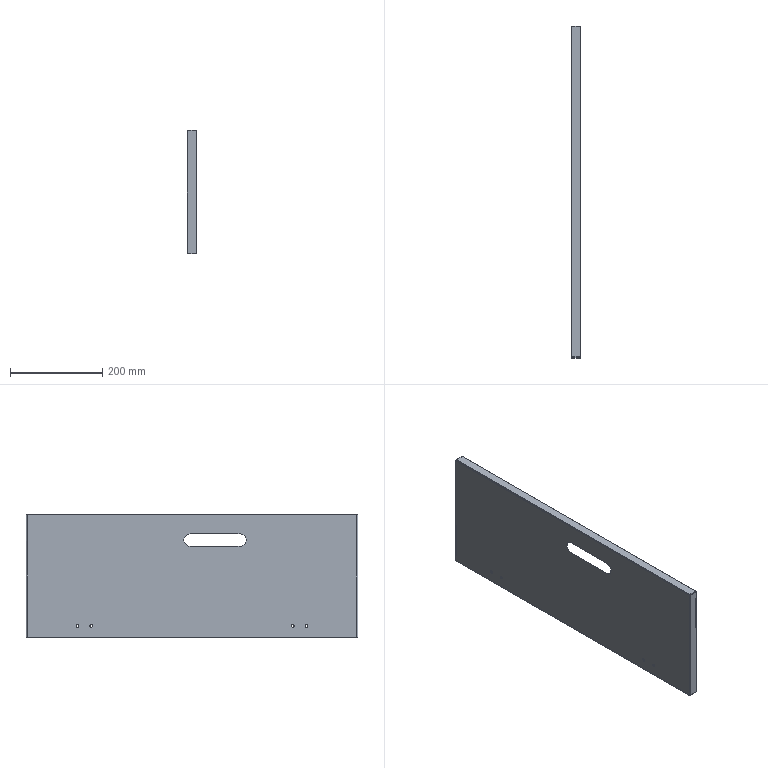Component | SolidWorks | FrameAssembly-1_SideDoor-1 | 1 solid | 82 faces | volume 313825 mm3 | plane 40 | cylinder 26 | spline 16 | commonest cylinder face diameters 6 x8 1.473 x8 3.873 x8 27 x2